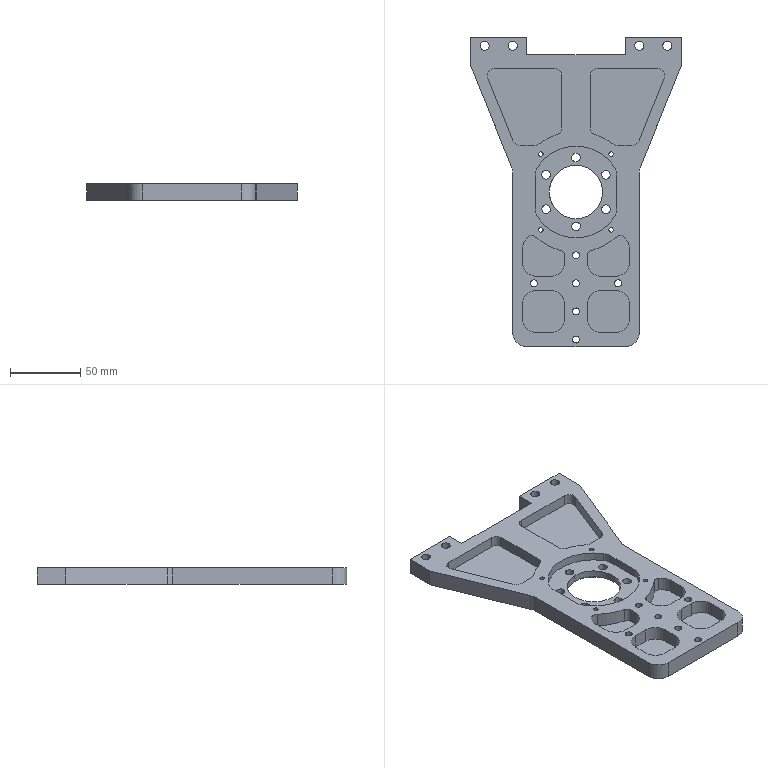CAM job | Mastercam | mm | 6 operations | part box 150 x 220 x 12
1. 2D High Speed (2D Area Mill) | 12 - 12 平铣刀
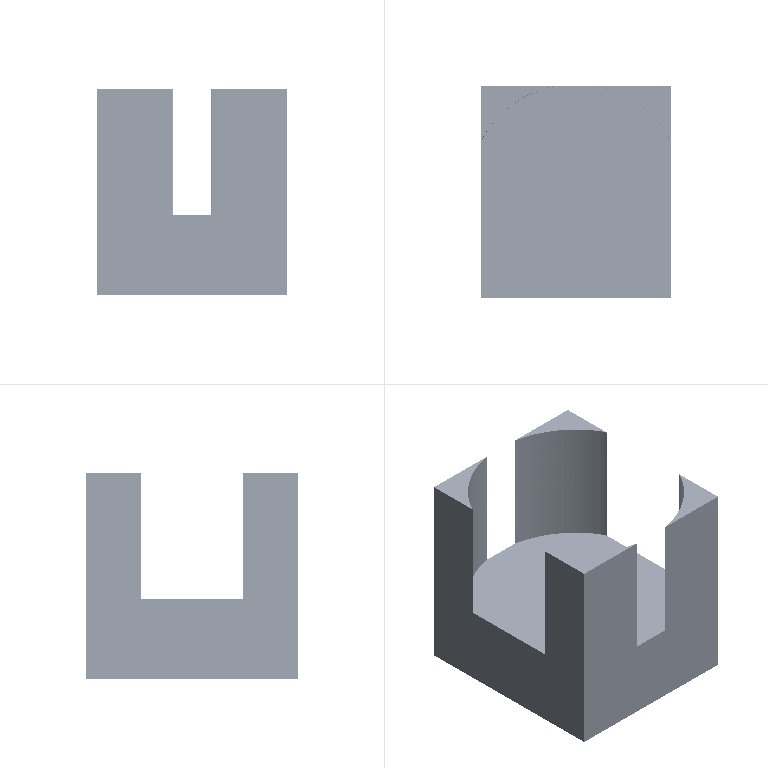2. Contour (2D) | 12 - 12 平铣刀
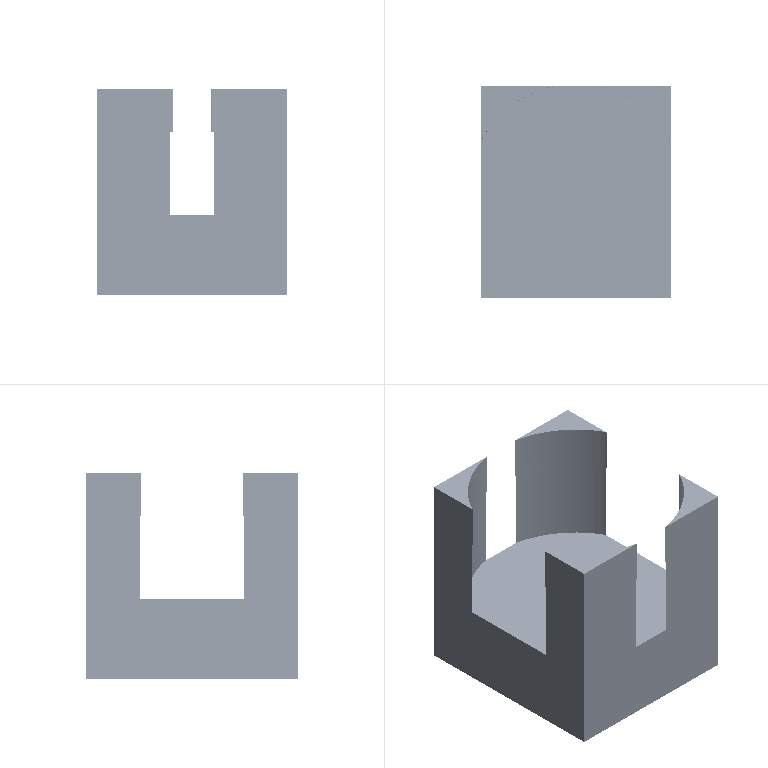3. Contour (Ramp) | 12 - 12 平铣刀
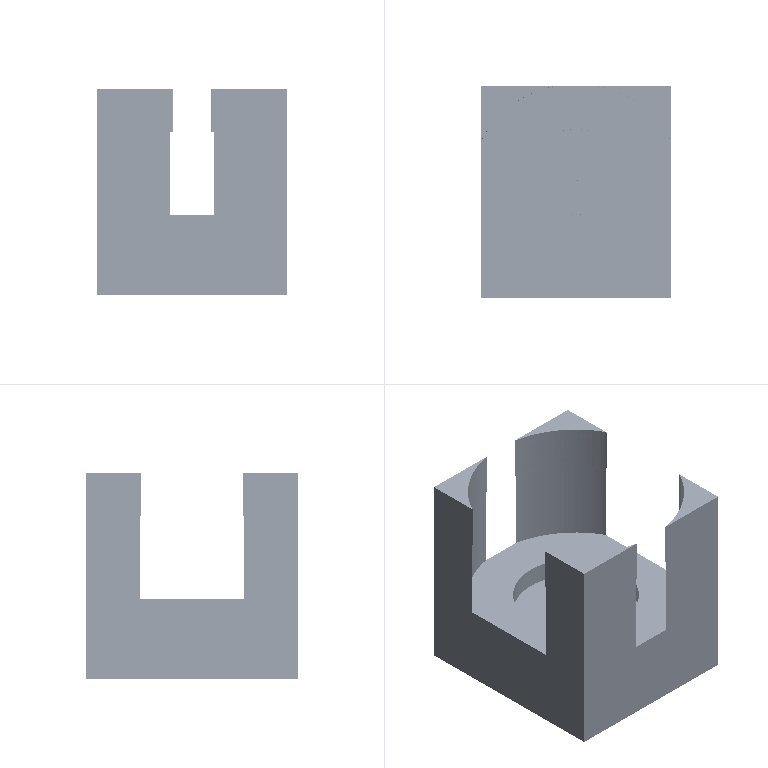4. Contour (2D) | 12 - 12 平铣刀
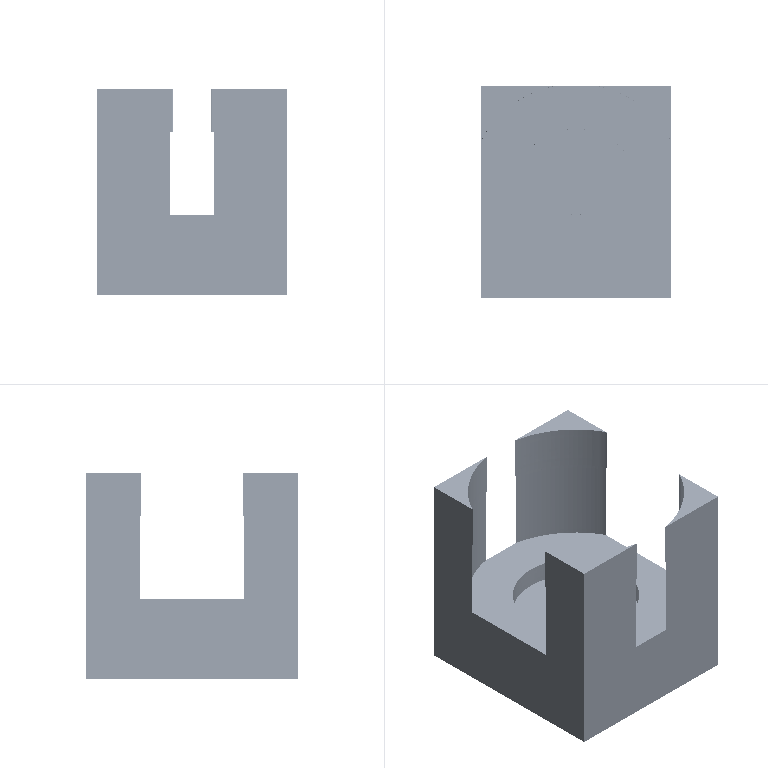5. Drill/Counterbore | 7 - 4 倒角刀
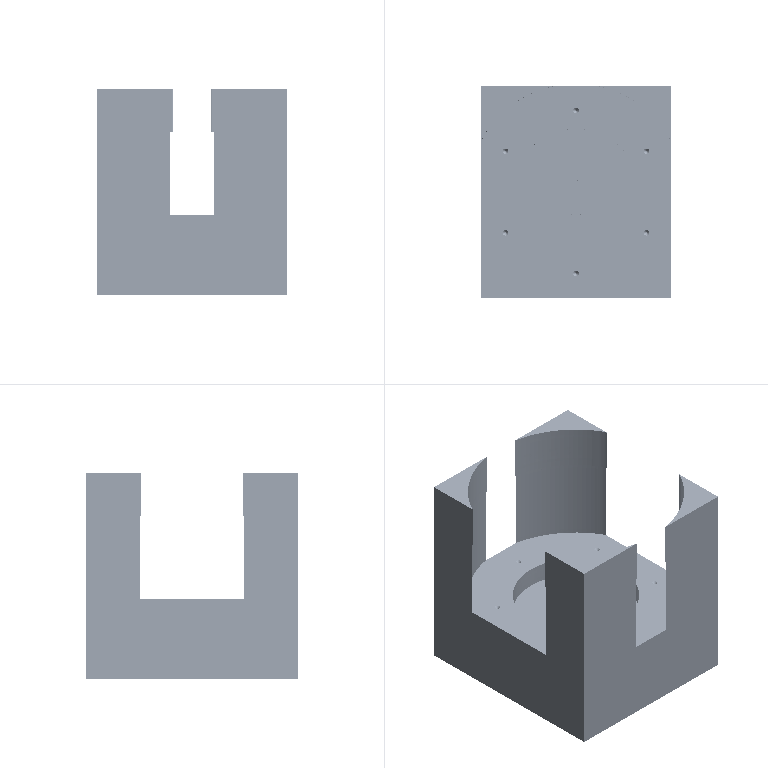6. Contour (2D chamfer) | 7 - 4 倒角刀